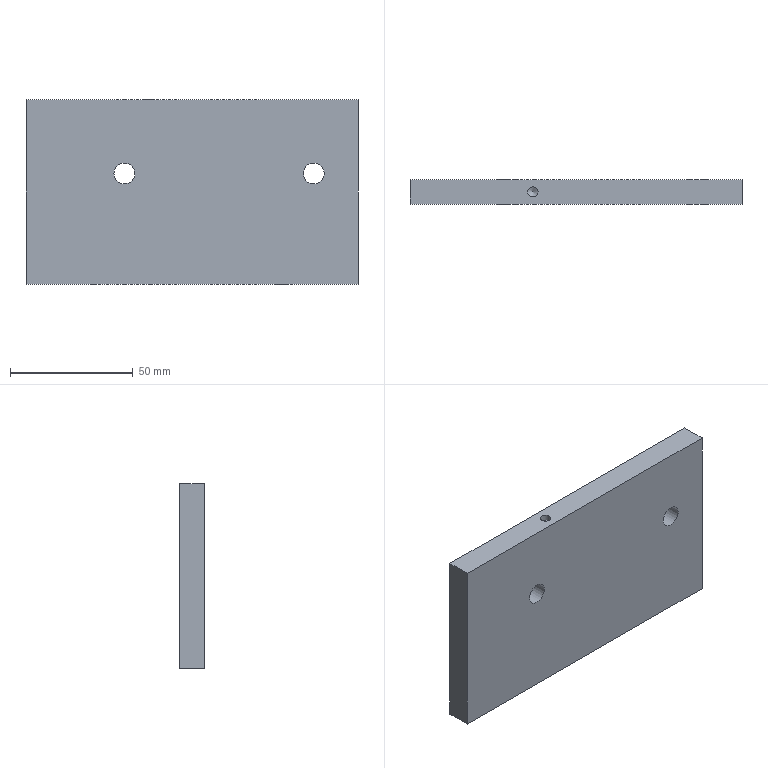Component | NX | FIXED_PLATE_15 | 1 solid | 14 faces | box 135 x 10 x 75 mm | volume 97868 mm3 | plane 6 | cylinder 5 | cone 3 | commonest cylinder face diameters 8.5 x2 6.8 x2 4.2 x1
STEP:
#1=CARTESIAN_POINT('',(0.,0.,0.));
#2=DIRECTION('',(0.,0.,1.));
#3=DIRECTION('',(1.,0.,0.));
#4=AXIS2_PLACEMENT_3D('',#1,#2,#3);
#5=CARTESIAN_POINT('',(1334.254,1421.,706.574));
#6=VERTEX_POINT('',#5);
#7=CARTESIAN_POINT('',(1334.254,1421.,781.574));
#8=VERTEX_POINT('',#7);
#9=CARTESIAN_POINT('',(1334.254,1421.,706.574));
#10=DIRECTION('',(0.,0.,1.));
#11=VECTOR('',#10,1.);
#12=LINE('',#9,#11);
#13=CARTESIAN_POINT('',(1334.254,1431.,706.574));
#14=DIRECTION('',(1.,0.,0.));
#15=DIRECTION('',(0.,0.,-1.));
#16=AXIS2_PLACEMENT_3D('',#13,#14,#15);
#17=PLANE('',#16);
#18=CARTESIAN_POINT('',(0.,-10.));
#19=DIRECTION('',(-1.,0.));
#20=VECTOR('',#19,1.);
#21=LINE('',#18,#20);
#22=(GEOMETRIC_REPRESENTATION_CONTEXT(2)PARAMETRIC_REPRESENTATION_CONTEXT()REPRESENTATION_CONTEXT('',''));
#23=DEFINITIONAL_REPRESENTATION('',(#21),#22);
#24=PCURVE('',#17,#23);
#25=CARTESIAN_POINT('',(1374.254,1421.,751.574));
#26=DIRECTION('',(0.,1.,0.));
#27=DIRECTION('',(0.,0.,1.));
#28=AXIS2_PLACEMENT_3D('',#25,#26,#27);
#29=PLANE('',#28);
#30=CARTESIAN_POINT('',(-45.,-40.));
#31=DIRECTION('',(1.,0.));
#32=VECTOR('',#31,1.);
#33=LINE('',#30,#32);
#34=(GEOMETRIC_REPRESENTATION_CONTEXT(2)PARAMETRIC_REPRESENTATION_CONTEXT()REPRESENTATION_CONTEXT('',''));
#35=DEFINITIONAL_REPRESENTATION('',(#33),#34);
#36=PCURVE('',#29,#35);
#37=SURFACE_CURVE('',#12,(#24,#36),.PCURVE_S1.);
#38=EDGE_CURVE('',#6,#8,#37,.T.);
#39=ORIENTED_EDGE('',*,*,#38,.T.);
#40=CARTESIAN_POINT('',(1334.254,1431.,781.574));
#41=VERTEX_POINT('',#40);
#42=CARTESIAN_POINT('',(1334.254,1431.,781.574));
#43=DIRECTION('',(0.,-1.,0.));
#44=VECTOR('',#43,1.);
#45=LINE('',#42,#44);
#46=CARTESIAN_POINT('',(-75.,0.));
#47=DIRECTION('',(0.,-1.));
#48=VECTOR('',#47,1.);
#49=LINE('',#46,#48);
#50=(GEOMETRIC_REPRESENTATION_CONTEXT(2)PARAMETRIC_REPRESENTATION_CONTEXT()REPRESENTATION_CONTEXT('',''));
#51=DEFINITIONAL_REPRESENTATION('',(#49),#50);
#52=PCURVE('',#17,#51);
#53=CARTESIAN_POINT('',(1334.254,1431.,781.574));
#54=DIRECTION('',(0.,0.,-1.));
#55=DIRECTION('',(-1.,0.,-0.));
#56=AXIS2_PLACEMENT_3D('',#53,#54,#55);
#57=PLANE('',#56);
#58=CARTESIAN_POINT('',(0.,0.));
#59=DIRECTION('',(0.,-1.));
#60=VECTOR('',#59,1.);
#61=LINE('',#58,#60);
#62=(GEOMETRIC_REPRESENTATION_CONTEXT(2)PARAMETRIC_REPRESENTATION_CONTEXT()REPRESENTATION_CONTEXT('',''));
#63=DEFINITIONAL_REPRESENTATION('',(#61),#62);
#64=PCURVE('',#57,#63);
#65=SURFACE_CURVE('',#45,(#52,#64),.PCURVE_S1.);
#66=EDGE_CURVE('',#41,#8,#65,.T.);
#67=ORIENTED_EDGE('',*,*,#66,.F.);
#68=CARTESIAN_POINT('',(1334.254,1431.,706.574));
#69=VERTEX_POINT('',#68);
#70=CARTESIAN_POINT('',(1334.254,1431.,706.574));
#71=DIRECTION('',(0.,0.,1.));
#72=VECTOR('',#71,1.);
#73=LINE('',#70,#72);
#74=CARTESIAN_POINT('',(0.,0.));
#75=DIRECTION('',(-1.,0.));
#76=VECTOR('',#75,1.);
#77=LINE('',#74,#76);
#78=(GEOMETRIC_REPRESENTATION_CONTEXT(2)PARAMETRIC_REPRESENTATION_CONTEXT()REPRESENTATION_CONTEXT('',''));
#79=DEFINITIONAL_REPRESENTATION('',(#77),#78);
#80=PCURVE('',#17,#79);
#81=CARTESIAN_POINT('',(1374.254,1431.,751.574));
#82=DIRECTION('',(0.,1.,0.));
#83=DIRECTION('',(0.,0.,1.));
#84=AXIS2_PLACEMENT_3D('',#81,#82,#83);
#85=PLANE('',#84);
#86=CARTESIAN_POINT('',(-45.,-40.));
#87=DIRECTION('',(1.,0.));
#88=VECTOR('',#87,1.);
#89=LINE('',#86,#88);
#90=(GEOMETRIC_REPRESENTATION_CONTEXT(2)PARAMETRIC_REPRESENTATION_CONTEXT()REPRESENTATION_CONTEXT('',''));
#91=DEFINITIONAL_REPRESENTATION('',(#89),#90);
#92=PCURVE('',#85,#91);
#93=SURFACE_CURVE('',#73,(#80,#92),.PCURVE_S1.);
#94=EDGE_CURVE('',#69,#41,#93,.T.);
#95=ORIENTED_EDGE('',*,*,#94,.F.);
#96=CARTESIAN_POINT('',(1334.254,1431.,706.574));
#97=DIRECTION('',(0.,-1.,0.));
#98=VECTOR('',#97,1.);
#99=LINE('',#96,#98);
#100=CARTESIAN_POINT('',(0.,0.));
#101=DIRECTION('',(0.,-1.));
#102=VECTOR('',#101,1.);
#103=LINE('',#100,#102);
#104=(GEOMETRIC_REPRESENTATION_CONTEXT(2)PARAMETRIC_REPRESENTATION_CONTEXT()REPRESENTATION_CONTEXT('',''));
#105=DEFINITIONAL_REPRESENTATION('',(#103),#104);
#106=PCURVE('',#17,#105);
#107=CARTESIAN_POINT('',(1469.254,1431.,706.574));
#108=DIRECTION('',(0.,0.,1.));
#109=DIRECTION('',(1.,0.,0.));
#110=AXIS2_PLACEMENT_3D('',#107,#108,#109);
#111=PLANE('',#110);
#112=CARTESIAN_POINT('',(-135.,0.));
#113=DIRECTION('',(0.,-1.));
#114=VECTOR('',#113,1.);
#115=LINE('',#112,#114);
#116=(GEOMETRIC_REPRESENTATION_CONTEXT(2)PARAMETRIC_REPRESENTATION_CONTEXT()REPRESENTATION_CONTEXT('',''));
#117=DEFINITIONAL_REPRESENTATION('',(#115),#116);
#118=PCURVE('',#111,#117);
#119=SURFACE_CURVE('',#99,(#106,#118),.PCURVE_S1.);
#120=EDGE_CURVE('',#69,#6,#119,.T.);
#121=ORIENTED_EDGE('',*,*,#120,.T.);
#122=EDGE_LOOP('',(#39,#67,#95,#121));
#123=FACE_BOUND('',#122,.T.);
#124=ADVANCED_FACE('',(#123),#17,.F.);
#125=CARTESIAN_POINT('',(1382.154,1426.,781.574));
#126=VERTEX_POINT('',#125);
#127=CARTESIAN_POINT('',(1384.254,1426.,781.574));
#128=DIRECTION('',(0.,0.,-1.));
#129=DIRECTION('',(-1.,0.,-0.));
#130=AXIS2_PLACEMENT_3D('',#127,#128,#129);
#131=CIRCLE('',#130,2.1);
#132=CARTESIAN_POINT('',(-50.,-5.));
#133=DIRECTION('',(1.,0.));
#134=AXIS2_PLACEMENT_2D('',#132,#133);
#135=CIRCLE('',#134,2.1);
#136=(GEOMETRIC_REPRESENTATION_CONTEXT(2)PARAMETRIC_REPRESENTATION_CONTEXT()REPRESENTATION_CONTEXT('',''));
#137=DEFINITIONAL_REPRESENTATION('',(#135),#136);
#138=PCURVE('',#57,#137);
#139=CARTESIAN_POINT('',(1384.254,1426.,781.574));
#140=DIRECTION('',(0.,0.,-1.));
#141=DIRECTION('',(-1.,0.,-0.));
#142=AXIS2_PLACEMENT_3D('',#139,#140,#141);
#143=CYLINDRICAL_SURFACE('',#142,2.1);
#144=CARTESIAN_POINT('',(0.,0.));
#145=DIRECTION('',(1.,0.));
#146=VECTOR('',#145,1.);
#147=LINE('',#144,#146);
#148=(GEOMETRIC_REPRESENTATION_CONTEXT(2)PARAMETRIC_REPRESENTATION_CONTEXT()REPRESENTATION_CONTEXT('',''));
#149=DEFINITIONAL_REPRESENTATION('',(#147),#148);
#150=PCURVE('',#143,#149);
#151=SURFACE_CURVE('',#131,(#138,#150),.PCURVE_S1.);
#152=EDGE_CURVE('',#126,#126,#151,.T.);
#153=ORIENTED_EDGE('',*,*,#152,.T.);
#154=EDGE_LOOP('',(#153));
#155=FACE_BOUND('',#154,.T.);
#156=CARTESIAN_POINT('',(1469.254,1421.,781.574));
#157=VERTEX_POINT('',#156);
#158=CARTESIAN_POINT('',(1334.254,1421.,781.574));
#159=DIRECTION('',(1.,0.,0.));
#160=VECTOR('',#159,1.);
#161=LINE('',#158,#160);
#162=CARTESIAN_POINT('',(0.,-10.));
#163=DIRECTION('',(-1.,0.));
#164=VECTOR('',#163,1.);
#165=LINE('',#162,#164);
#166=(GEOMETRIC_REPRESENTATION_CONTEXT(2)PARAMETRIC_REPRESENTATION_CONTEXT()REPRESENTATION_CONTEXT('',''));
#167=DEFINITIONAL_REPRESENTATION('',(#165),#166);
#168=PCURVE('',#57,#167);
#169=CARTESIAN_POINT('',(30.,-40.));
#170=DIRECTION('',(0.,1.));
#171=VECTOR('',#170,1.);
#172=LINE('',#169,#171);
#173=(GEOMETRIC_REPRESENTATION_CONTEXT(2)PARAMETRIC_REPRESENTATION_CONTEXT()REPRESENTATION_CONTEXT('',''));
#174=DEFINITIONAL_REPRESENTATION('',(#172),#173);
#175=PCURVE('',#29,#174);
#176=SURFACE_CURVE('',#161,(#168,#175),.PCURVE_S1.);
#177=EDGE_CURVE('',#8,#157,#176,.T.);
#178=ORIENTED_EDGE('',*,*,#177,.T.);
#179=CARTESIAN_POINT('',(1469.254,1431.,781.574));
#180=VERTEX_POINT('',#179);
#181=CARTESIAN_POINT('',(1469.254,1431.,781.574));
#182=DIRECTION('',(0.,-1.,0.));
#183=VECTOR('',#182,1.);
#184=LINE('',#181,#183);
#185=CARTESIAN_POINT('',(-135.,0.));
#186=DIRECTION('',(0.,-1.));
#187=VECTOR('',#186,1.);
#188=LINE('',#185,#187);
#189=(GEOMETRIC_REPRESENTATION_CONTEXT(2)PARAMETRIC_REPRESENTATION_CONTEXT()REPRESENTATION_CONTEXT('',''));
#190=DEFINITIONAL_REPRESENTATION('',(#188),#189);
#191=PCURVE('',#57,#190);
#192=CARTESIAN_POINT('',(1469.254,1431.,781.574));
#193=DIRECTION('',(-1.,0.,0.));
#194=DIRECTION('',(0.,0.,1.));
#195=AXIS2_PLACEMENT_3D('',#192,#193,#194);
#196=PLANE('',#195);
#197=CARTESIAN_POINT('',(0.,0.));
#198=DIRECTION('',(0.,-1.));
#199=VECTOR('',#198,1.);
#200=LINE('',#197,#199);
#201=(GEOMETRIC_REPRESENTATION_CONTEXT(2)PARAMETRIC_REPRESENTATION_CONTEXT()REPRESENTATION_CONTEXT('',''));
#202=DEFINITIONAL_REPRESENTATION('',(#200),#201);
#203=PCURVE('',#196,#202);
#204=SURFACE_CURVE('',#184,(#191,#203),.PCURVE_S1.);
#205=EDGE_CURVE('',#180,#157,#204,.T.);
#206=ORIENTED_EDGE('',*,*,#205,.F.);
#207=CARTESIAN_POINT('',(1334.254,1431.,781.574));
#208=DIRECTION('',(1.,0.,0.));
#209=VECTOR('',#208,1.);
#210=LINE('',#207,#209);
#211=CARTESIAN_POINT('',(0.,0.));
#212=DIRECTION('',(-1.,0.));
#213=VECTOR('',#212,1.);
#214=LINE('',#211,#213);
#215=(GEOMETRIC_REPRESENTATION_CONTEXT(2)PARAMETRIC_REPRESENTATION_CONTEXT()REPRESENTATION_CONTEXT('',''));
#216=DEFINITIONAL_REPRESENTATION('',(#214),#215);
#217=PCURVE('',#57,#216);
#218=CARTESIAN_POINT('',(30.,-40.));
#219=DIRECTION('',(0.,1.));
#220=VECTOR('',#219,1.);
#221=LINE('',#218,#220);
#222=(GEOMETRIC_REPRESENTATION_CONTEXT(2)PARAMETRIC_REPRESENTATION_CONTEXT()REPRESENTATION_CONTEXT('',''));
#223=DEFINITIONAL_REPRESENTATION('',(#221),#222);
#224=PCURVE('',#85,#223);
#225=SURFACE_CURVE('',#210,(#217,#224),.PCURVE_S1.);
#226=EDGE_CURVE('',#41,#180,#225,.T.);
#227=ORIENTED_EDGE('',*,*,#226,.F.);
#228=ORIENTED_EDGE('',*,*,#66,.T.);
#229=EDGE_LOOP('',(#178,#206,#227,#228));
#230=FACE_BOUND('',#229,.T.);
#231=ADVANCED_FACE('',(#155,#230),#57,.F.);
#232=CARTESIAN_POINT('',(1469.254,1421.,706.574));
#233=VERTEX_POINT('',#232);
#234=CARTESIAN_POINT('',(1469.254,1421.,781.574));
#235=DIRECTION('',(0.,0.,-1.));
#236=VECTOR('',#235,1.);
#237=LINE('',#234,#236);
#238=CARTESIAN_POINT('',(0.,-10.));
#239=DIRECTION('',(-1.,0.));
#240=VECTOR('',#239,1.);
#241=LINE('',#238,#240);
#242=(GEOMETRIC_REPRESENTATION_CONTEXT(2)PARAMETRIC_REPRESENTATION_CONTEXT()REPRESENTATION_CONTEXT('',''));
#243=DEFINITIONAL_REPRESENTATION('',(#241),#242);
#244=PCURVE('',#196,#243);
#245=CARTESIAN_POINT('',(30.,95.));
#246=DIRECTION('',(-1.,0.));
#247=VECTOR('',#246,1.);
#248=LINE('',#245,#247);
#249=(GEOMETRIC_REPRESENTATION_CONTEXT(2)PARAMETRIC_REPRESENTATION_CONTEXT()REPRESENTATION_CONTEXT('',''));
#250=DEFINITIONAL_REPRESENTATION('',(#248),#249);
#251=PCURVE('',#29,#250);
#252=SURFACE_CURVE('',#237,(#244,#251),.PCURVE_S1.);
#253=EDGE_CURVE('',#157,#233,#252,.T.);
#254=ORIENTED_EDGE('',*,*,#253,.T.);
#255=CARTESIAN_POINT('',(1469.254,1431.,706.574));
#256=VERTEX_POINT('',#255);
#257=CARTESIAN_POINT('',(1469.254,1431.,706.574));
#258=DIRECTION('',(0.,-1.,0.));
#259=VECTOR('',#258,1.);
#260=LINE('',#257,#259);
#261=CARTESIAN_POINT('',(-75.,0.));
#262=DIRECTION('',(0.,-1.));
#263=VECTOR('',#262,1.);
#264=LINE('',#261,#263);
#265=(GEOMETRIC_REPRESENTATION_CONTEXT(2)PARAMETRIC_REPRESENTATION_CONTEXT()REPRESENTATION_CONTEXT('',''));
#266=DEFINITIONAL_REPRESENTATION('',(#264),#265);
#267=PCURVE('',#196,#266);
#268=CARTESIAN_POINT('',(0.,0.));
#269=DIRECTION('',(0.,-1.));
#270=VECTOR('',#269,1.);
#271=LINE('',#268,#270);
#272=(GEOMETRIC_REPRESENTATION_CONTEXT(2)PARAMETRIC_REPRESENTATION_CONTEXT()REPRESENTATION_CONTEXT('',''));
#273=DEFINITIONAL_REPRESENTATION('',(#271),#272);
#274=PCURVE('',#111,#273);
#275=SURFACE_CURVE('',#260,(#267,#274),.PCURVE_S1.);
#276=EDGE_CURVE('',#256,#233,#275,.T.);
#277=ORIENTED_EDGE('',*,*,#276,.F.);
#278=CARTESIAN_POINT('',(1469.254,1431.,781.574));
#279=DIRECTION('',(0.,0.,-1.));
#280=VECTOR('',#279,1.);
#281=LINE('',#278,#280);
#282=CARTESIAN_POINT('',(0.,0.));
#283=DIRECTION('',(-1.,0.));
#284=VECTOR('',#283,1.);
#285=LINE('',#282,#284);
#286=(GEOMETRIC_REPRESENTATION_CONTEXT(2)PARAMETRIC_REPRESENTATION_CONTEXT()REPRESENTATION_CONTEXT('',''));
#287=DEFINITIONAL_REPRESENTATION('',(#285),#286);
#288=PCURVE('',#196,#287);
#289=CARTESIAN_POINT('',(30.,95.));
#290=DIRECTION('',(-1.,0.));
#291=VECTOR('',#290,1.);
#292=LINE('',#289,#291);
#293=(GEOMETRIC_REPRESENTATION_CONTEXT(2)PARAMETRIC_REPRESENTATION_CONTEXT()REPRESENTATION_CONTEXT('',''));
#294=DEFINITIONAL_REPRESENTATION('',(#292),#293);
#295=PCURVE('',#85,#294);
#296=SURFACE_CURVE('',#281,(#288,#295),.PCURVE_S1.);
#297=EDGE_CURVE('',#180,#256,#296,.T.);
#298=ORIENTED_EDGE('',*,*,#297,.F.);
#299=ORIENTED_EDGE('',*,*,#205,.T.);
#300=EDGE_LOOP('',(#254,#277,#298,#299));
#301=FACE_BOUND('',#300,.T.);
#302=ADVANCED_FACE('',(#301),#196,.F.);
#303=CARTESIAN_POINT('',(1378.504,1431.,751.574));
#304=VERTEX_POINT('',#303);
#305=CARTESIAN_POINT('',(1374.254,1431.,751.574));
#306=DIRECTION('',(0.,1.,0.));
#307=DIRECTION('',(1.,0.,0.));
#308=AXIS2_PLACEMENT_3D('',#305,#306,#307);
#309=CIRCLE('',#308,4.25);
#310=CARTESIAN_POINT('',(1374.254,1431.,751.574));
#311=DIRECTION('',(0.,-1.,0.));
#312=DIRECTION('',(0.,0.,-1.));
#313=AXIS2_PLACEMENT_3D('',#310,#311,#312);
#314=CYLINDRICAL_SURFACE('',#313,4.25);
#315=CARTESIAN_POINT('',(7.854,0.));
#316=DIRECTION('',(-1.,0.));
#317=VECTOR('',#316,1.);
#318=LINE('',#315,#317);
#319=(GEOMETRIC_REPRESENTATION_CONTEXT(2)PARAMETRIC_REPRESENTATION_CONTEXT()REPRESENTATION_CONTEXT('',''));
#320=DEFINITIONAL_REPRESENTATION('',(#318),#319);
#321=PCURVE('',#314,#320);
#322=CARTESIAN_POINT('',(0.,0.));
#323=DIRECTION('',(0.,1.));
#324=AXIS2_PLACEMENT_2D('',#322,#323);
#325=CIRCLE('',#324,4.25);
#326=(GEOMETRIC_REPRESENTATION_CONTEXT(2)PARAMETRIC_REPRESENTATION_CONTEXT()REPRESENTATION_CONTEXT('',''));
#327=DEFINITIONAL_REPRESENTATION('',(#325),#326);
#328=PCURVE('',#85,#327);
#329=SURFACE_CURVE('',#309,(#321,#328),.PCURVE_S1.);
#330=EDGE_CURVE('',#304,#304,#329,.T.);
#331=ORIENTED_EDGE('',*,*,#330,.F.);
#332=CARTESIAN_POINT('',(1378.504,1421.,751.574));
#333=VERTEX_POINT('',#332);
#334=CARTESIAN_POINT('',(1378.504,1431.,751.574));
#335=CARTESIAN_POINT('',(1378.504,1421.,751.574));
#336=B_SPLINE_CURVE_WITH_KNOTS('',1,(#334,#335),.UNSPECIFIED.,.F.,.F.,(2,2),(0.,10.),.PIECEWISE_BEZIER_KNOTS.);
#337=CARTESIAN_POINT('',(7.854,0.));
#338=DIRECTION('',(0.,1.));
#339=VECTOR('',#338,1.);
#340=LINE('',#337,#339);
#341=(GEOMETRIC_REPRESENTATION_CONTEXT(2)PARAMETRIC_REPRESENTATION_CONTEXT()REPRESENTATION_CONTEXT('',''));
#342=DEFINITIONAL_REPRESENTATION('',(#340),#341);
#343=PCURVE('',#314,#342);
#344=CARTESIAN_POINT('',(1.571,0.));
#345=DIRECTION('',(0.,1.));
#346=VECTOR('',#345,1.);
#347=LINE('',#344,#346);
#348=(GEOMETRIC_REPRESENTATION_CONTEXT(2)PARAMETRIC_REPRESENTATION_CONTEXT()REPRESENTATION_CONTEXT('',''));
#349=DEFINITIONAL_REPRESENTATION('',(#347),#348);
#350=PCURVE('',#314,#349);
#351=SEAM_CURVE('',#336,(#343,#350),.PCURVE_S1.);
#352=EDGE_CURVE('',#304,#333,#351,.T.);
#353=ORIENTED_EDGE('',*,*,#352,.T.);
#354=CARTESIAN_POINT('',(1374.254,1421.,751.574));
#355=DIRECTION('',(0.,1.,0.));
#356=DIRECTION('',(1.,0.,0.));
#357=AXIS2_PLACEMENT_3D('',#354,#355,#356);
#358=CIRCLE('',#357,4.25);
#359=CARTESIAN_POINT('',(7.854,10.));
#360=DIRECTION('',(-1.,0.));
#361=VECTOR('',#360,1.);
#362=LINE('',#359,#361);
#363=(GEOMETRIC_REPRESENTATION_CONTEXT(2)PARAMETRIC_REPRESENTATION_CONTEXT()REPRESENTATION_CONTEXT('',''));
#364=DEFINITIONAL_REPRESENTATION('',(#362),#363);
#365=PCURVE('',#314,#364);
#366=CARTESIAN_POINT('',(0.,0.));
#367=DIRECTION('',(0.,1.));
#368=AXIS2_PLACEMENT_2D('',#366,#367);
#369=CIRCLE('',#368,4.25);
#370=(GEOMETRIC_REPRESENTATION_CONTEXT(2)PARAMETRIC_REPRESENTATION_CONTEXT()REPRESENTATION_CONTEXT('',''));
#371=DEFINITIONAL_REPRESENTATION('',(#369),#370);
#372=PCURVE('',#29,#371);
#373=SURFACE_CURVE('',#358,(#365,#372),.PCURVE_S1.);
#374=EDGE_CURVE('',#333,#333,#373,.T.);
#375=ORIENTED_EDGE('',*,*,#374,.T.);
#376=ORIENTED_EDGE('',*,*,#352,.F.);
#377=EDGE_LOOP('',(#331,#353,#375,#376));
#378=FACE_BOUND('',#377,.F.);
#379=ADVANCED_FACE('',(#378),#314,.F.);
#380=CARTESIAN_POINT('',(1442.654,1427.,706.574));
#381=VERTEX_POINT('',#380);
#382=CARTESIAN_POINT('',(1439.254,1427.,706.574));
#383=DIRECTION('',(0.,0.,1.));
#384=DIRECTION('',(1.,0.,0.));
#385=AXIS2_PLACEMENT_3D('',#382,#383,#384);
#386=CIRCLE('',#385,3.4);
#387=CARTESIAN_POINT('',(-30.,-4.));
#388=DIRECTION('',(1.,0.));
#389=AXIS2_PLACEMENT_2D('',#387,#388);
#390=CIRCLE('',#389,3.4);
#391=(GEOMETRIC_REPRESENTATION_CONTEXT(2)PARAMETRIC_REPRESENTATION_CONTEXT()REPRESENTATION_CONTEXT('',''));
#392=DEFINITIONAL_REPRESENTATION('',(#390),#391);
#393=PCURVE('',#111,#392);
#394=CARTESIAN_POINT('',(1439.254,1427.,706.574));
#395=DIRECTION('',(0.,0.,1.));
#396=DIRECTION('',(1.,0.,0.));
#397=AXIS2_PLACEMENT_3D('',#394,#395,#396);
#398=CYLINDRICAL_SURFACE('',#397,3.4);
#399=CARTESIAN_POINT('',(0.,0.));
#400=DIRECTION('',(1.,0.));
#401=VECTOR('',#400,1.);
#402=LINE('',#399,#401);
#403=(GEOMETRIC_REPRESENTATION_CONTEXT(2)PARAMETRIC_REPRESENTATION_CONTEXT()REPRESENTATION_CONTEXT('',''));
#404=DEFINITIONAL_REPRESENTATION('',(#402),#403);
#405=PCURVE('',#398,#404);
#406=SURFACE_CURVE('',#386,(#393,#405),.PCURVE_S1.);
#407=EDGE_CURVE('',#381,#381,#406,.T.);
#408=ORIENTED_EDGE('',*,*,#407,.T.);
#409=EDGE_LOOP('',(#408));
#410=FACE_BOUND('',#409,.T.);
#411=CARTESIAN_POINT('',(1367.654,1427.,706.574));
#412=VERTEX_POINT('',#411);
#413=CARTESIAN_POINT('',(1364.254,1427.,706.574));
#414=DIRECTION('',(0.,0.,1.));
#415=DIRECTION('',(1.,0.,0.));
#416=AXIS2_PLACEMENT_3D('',#413,#414,#415);
#417=CIRCLE('',#416,3.4);
#418=CARTESIAN_POINT('',(-105.,-4.));
#419=DIRECTION('',(1.,0.));
#420=AXIS2_PLACEMENT_2D('',#418,#419);
#421=CIRCLE('',#420,3.4);
#422=(GEOMETRIC_REPRESENTATION_CONTEXT(2)PARAMETRIC_REPRESENTATION_CONTEXT()REPRESENTATION_CONTEXT('',''));
#423=DEFINITIONAL_REPRESENTATION('',(#421),#422);
#424=PCURVE('',#111,#423);
#425=CARTESIAN_POINT('',(1364.254,1427.,706.574));
#426=DIRECTION('',(0.,0.,1.));
#427=DIRECTION('',(1.,0.,0.));
#428=AXIS2_PLACEMENT_3D('',#425,#426,#427);
#429=CYLINDRICAL_SURFACE('',#428,3.4);
#430=CARTESIAN_POINT('',(0.,0.));
#431=DIRECTION('',(1.,0.));
#432=VECTOR('',#431,1.);
#433=LINE('',#430,#432);
#434=(GEOMETRIC_REPRESENTATION_CONTEXT(2)PARAMETRIC_REPRESENTATION_CONTEXT()REPRESENTATION_CONTEXT('',''));
#435=DEFINITIONAL_REPRESENTATION('',(#433),#434);
#436=PCURVE('',#429,#435);
#437=SURFACE_CURVE('',#417,(#424,#436),.PCURVE_S1.);
#438=EDGE_CURVE('',#412,#412,#437,.T.);
#439=ORIENTED_EDGE('',*,*,#438,.T.);
#440=EDGE_LOOP('',(#439));
#441=FACE_BOUND('',#440,.T.);
#442=CARTESIAN_POINT('',(1469.254,1421.,706.574));
#443=DIRECTION('',(-1.,0.,0.));
#444=VECTOR('',#443,1.);
#445=LINE('',#442,#444);
#446=CARTESIAN_POINT('',(0.,-10.));
#447=DIRECTION('',(-1.,0.));
#448=VECTOR('',#447,1.);
#449=LINE('',#446,#448);
#450=(GEOMETRIC_REPRESENTATION_CONTEXT(2)PARAMETRIC_REPRESENTATION_CONTEXT()REPRESENTATION_CONTEXT('',''));
#451=DEFINITIONAL_REPRESENTATION('',(#449),#450);
#452=PCURVE('',#111,#451);
#453=CARTESIAN_POINT('',(-45.,95.));
#454=DIRECTION('',(0.,-1.));
#455=VECTOR('',#454,1.);
#456=LINE('',#453,#455);
#457=(GEOMETRIC_REPRESENTATION_CONTEXT(2)PARAMETRIC_REPRESENTATION_CONTEXT()REPRESENTATION_CONTEXT('',''));
#458=DEFINITIONAL_REPRESENTATION('',(#456),#457);
#459=PCURVE('',#29,#458);
#460=SURFACE_CURVE('',#445,(#452,#459),.PCURVE_S1.);
#461=EDGE_CURVE('',#233,#6,#460,.T.);
#462=ORIENTED_EDGE('',*,*,#461,.T.);
#463=ORIENTED_EDGE('',*,*,#120,.F.);
#464=CARTESIAN_POINT('',(1469.254,1431.,706.574));
#465=DIRECTION('',(-1.,0.,0.));
#466=VECTOR('',#465,1.);
#467=LINE('',#464,#466);
#468=CARTESIAN_POINT('',(0.,0.));
#469=DIRECTION('',(-1.,0.));
#470=VECTOR('',#469,1.);
#471=LINE('',#468,#470);
#472=(GEOMETRIC_REPRESENTATION_CONTEXT(2)PARAMETRIC_REPRESENTATION_CONTEXT()REPRESENTATION_CONTEXT('',''));
#473=DEFINITIONAL_REPRESENTATION('',(#471),#472);
#474=PCURVE('',#111,#473);
#475=CARTESIAN_POINT('',(-45.,95.));
#476=DIRECTION('',(0.,-1.));
#477=VECTOR('',#476,1.);
#478=LINE('',#475,#477);
#479=(GEOMETRIC_REPRESENTATION_CONTEXT(2)PARAMETRIC_REPRESENTATION_CONTEXT()REPRESENTATION_CONTEXT('',''));
#480=DEFINITIONAL_REPRESENTATION('',(#478),#479);
#481=PCURVE('',#85,#480);
#482=SURFACE_CURVE('',#467,(#474,#481),.PCURVE_S1.);
#483=EDGE_CURVE('',#256,#69,#482,.T.);
#484=ORIENTED_EDGE('',*,*,#483,.F.);
#485=ORIENTED_EDGE('',*,*,#276,.T.);
#486=EDGE_LOOP('',(#462,#463,#484,#485));
#487=FACE_BOUND('',#486,.T.);
#488=ADVANCED_FACE('',(#410,#441,#487),#111,.F.);
#489=CARTESIAN_POINT('',(1455.504,1431.,751.574));
#490=VERTEX_POINT('',#489);
#491=CARTESIAN_POINT('',(1451.254,1431.,751.574));
#492=DIRECTION('',(0.,1.,0.));
#493=DIRECTION('',(1.,0.,0.));
#494=AXIS2_PLACEMENT_3D('',#491,#492,#493);
#495=CIRCLE('',#494,4.25);
#496=CARTESIAN_POINT('',(1451.254,1431.,751.574));
#497=DIRECTION('',(0.,-1.,0.));
#498=DIRECTION('',(0.,0.,-1.));
#499=AXIS2_PLACEMENT_3D('',#496,#497,#498);
#500=CYLINDRICAL_SURFACE('',#499,4.25);
#501=CARTESIAN_POINT('',(7.854,0.));
#502=DIRECTION('',(-1.,0.));
#503=VECTOR('',#502,1.);
#504=LINE('',#501,#503);
#505=(GEOMETRIC_REPRESENTATION_CONTEXT(2)PARAMETRIC_REPRESENTATION_CONTEXT()REPRESENTATION_CONTEXT('',''));
#506=DEFINITIONAL_REPRESENTATION('',(#504),#505);
#507=PCURVE('',#500,#506);
#508=CARTESIAN_POINT('',(0.,77.));
#509=DIRECTION('',(0.,1.));
#510=AXIS2_PLACEMENT_2D('',#508,#509);
#511=CIRCLE('',#510,4.25);
#512=(GEOMETRIC_REPRESENTATION_CONTEXT(2)PARAMETRIC_REPRESENTATION_CONTEXT()REPRESENTATION_CONTEXT('',''));
#513=DEFINITIONAL_REPRESENTATION('',(#511),#512);
#514=PCURVE('',#85,#513);
#515=SURFACE_CURVE('',#495,(#507,#514),.PCURVE_S1.);
#516=EDGE_CURVE('',#490,#490,#515,.T.);
#517=ORIENTED_EDGE('',*,*,#516,.F.);
#518=CARTESIAN_POINT('',(1455.504,1421.,751.574));
#519=VERTEX_POINT('',#518);
#520=CARTESIAN_POINT('',(1455.504,1431.,751.574));
#521=CARTESIAN_POINT('',(1455.504,1421.,751.574));
#522=B_SPLINE_CURVE_WITH_KNOTS('',1,(#520,#521),.UNSPECIFIED.,.F.,.F.,(2,2),(0.,10.),.PIECEWISE_BEZIER_KNOTS.);
#523=CARTESIAN_POINT('',(7.854,0.));
#524=DIRECTION('',(0.,1.));
#525=VECTOR('',#524,1.);
#526=LINE('',#523,#525);
#527=(GEOMETRIC_REPRESENTATION_CONTEXT(2)PARAMETRIC_REPRESENTATION_CONTEXT()REPRESENTATION_CONTEXT('',''));
#528=DEFINITIONAL_REPRESENTATION('',(#526),#527);
#529=PCURVE('',#500,#528);
#530=CARTESIAN_POINT('',(1.571,0.));
#531=DIRECTION('',(0.,1.));
#532=VECTOR('',#531,1.);
#533=LINE('',#530,#532);
#534=(GEOMETRIC_REPRESENTATION_CONTEXT(2)PARAMETRIC_REPRESENTATION_CONTEXT()REPRESENTATION_CONTEXT('',''));
#535=DEFINITIONAL_REPRESENTATION('',(#533),#534);
#536=PCURVE('',#500,#535);
#537=SEAM_CURVE('',#522,(#529,#536),.PCURVE_S1.);
#538=EDGE_CURVE('',#490,#519,#537,.T.);
#539=ORIENTED_EDGE('',*,*,#538,.T.);
#540=CARTESIAN_POINT('',(1451.254,1421.,751.574));
#541=DIRECTION('',(0.,1.,0.));
#542=DIRECTION('',(1.,0.,0.));
#543=AXIS2_PLACEMENT_3D('',#540,#541,#542);
#544=CIRCLE('',#543,4.25);
#545=CARTESIAN_POINT('',(7.854,10.));
#546=DIRECTION('',(-1.,0.));
#547=VECTOR('',#546,1.);
#548=LINE('',#545,#547);
#549=(GEOMETRIC_REPRESENTATION_CONTEXT(2)PARAMETRIC_REPRESENTATION_CONTEXT()REPRESENTATION_CONTEXT('',''));
#550=DEFINITIONAL_REPRESENTATION('',(#548),#549);
#551=PCURVE('',#500,#550);
#552=CARTESIAN_POINT('',(0.,77.));
#553=DIRECTION('',(0.,1.));
#554=AXIS2_PLACEMENT_2D('',#552,#553);
#555=CIRCLE('',#554,4.25);
#556=(GEOMETRIC_REPRESENTATION_CONTEXT(2)PARAMETRIC_REPRESENTATION_CONTEXT()REPRESENTATION_CONTEXT('',''));
#557=DEFINITIONAL_REPRESENTATION('',(#555),#556);
#558=PCURVE('',#29,#557);
#559=SURFACE_CURVE('',#544,(#551,#558),.PCURVE_S1.);
#560=EDGE_CURVE('',#519,#519,#559,.T.);
#561=ORIENTED_EDGE('',*,*,#560,.T.);
#562=ORIENTED_EDGE('',*,*,#538,.F.);
#563=EDGE_LOOP('',(#517,#539,#561,#562));
#564=FACE_BOUND('',#563,.F.);
#565=ADVANCED_FACE('',(#564),#500,.F.);
#566=ORIENTED_EDGE('',*,*,#94,.T.);
#567=ORIENTED_EDGE('',*,*,#226,.T.);
#568=ORIENTED_EDGE('',*,*,#297,.T.);
#569=ORIENTED_EDGE('',*,*,#483,.T.);
#570=EDGE_LOOP('',(#566,#567,#568,#569));
#571=FACE_BOUND('',#570,.T.);
#572=ORIENTED_EDGE('',*,*,#330,.F.);
#573=EDGE_LOOP('',(#572));
#574=FACE_BOUND('',#573,.T.);
#575=ORIENTED_EDGE('',*,*,#516,.F.);
#576=EDGE_LOOP('',(#575));
#577=FACE_BOUND('',#576,.T.);
#578=ADVANCED_FACE('',(#571,#574,#577),#85,.T.);
#579=ORIENTED_EDGE('',*,*,#38,.F.);
#580=ORIENTED_EDGE('',*,*,#461,.F.);
#581=ORIENTED_EDGE('',*,*,#253,.F.);
#582=ORIENTED_EDGE('',*,*,#177,.F.);
#583=EDGE_LOOP('',(#579,#580,#581,#582));
#584=FACE_BOUND('',#583,.T.);
#585=ORIENTED_EDGE('',*,*,#374,.T.);
#586=EDGE_LOOP('',(#585));
#587=FACE_BOUND('',#586,.T.);
#588=ORIENTED_EDGE('',*,*,#560,.T.);
#589=EDGE_LOOP('',(#588));
#590=FACE_BOUND('',#589,.T.);
#591=ADVANCED_FACE('',(#584,#587,#590),#29,.F.);
#592=CARTESIAN_POINT('',(1386.354,1426.,779.174));
#593=VERTEX_POINT('',#592);
#594=CARTESIAN_POINT('',(1382.154,1426.,779.174));
#595=VERTEX_POINT('',#594);
#596=CARTESIAN_POINT('',(1384.254,1426.,779.174));
#597=DIRECTION('',(-0.,0.,1.));
#598=DIRECTION('',(-1.,0.,-0.));
#599=AXIS2_PLACEMENT_3D('',#596,#597,#598);
#600=CIRCLE('',#599,2.1);
#601=CARTESIAN_POINT('',(1384.254,1426.,779.174));
#602=DIRECTION('',(-0.,0.,1.));
#603=DIRECTION('',(1.,0.,0.));
#604=AXIS2_PLACEMENT_3D('',#601,#602,#603);
#605=CONICAL_SURFACE('',#604,2.1,1.047);
#606=CARTESIAN_POINT('',(-3.142,-0.));
#607=DIRECTION('',(1.,0.));
#608=VECTOR('',#607,1.);
#609=LINE('',#606,#608);
#610=(GEOMETRIC_REPRESENTATION_CONTEXT(2)PARAMETRIC_REPRESENTATION_CONTEXT()REPRESENTATION_CONTEXT('',''));
#611=DEFINITIONAL_REPRESENTATION('',(#609),#610);
#612=PCURVE('',#605,#611);
#613=CARTESIAN_POINT('',(6.283,2.4));
#614=DIRECTION('',(-1.,0.));
#615=VECTOR('',#614,1.);
#616=LINE('',#613,#615);
#617=(GEOMETRIC_REPRESENTATION_CONTEXT(2)PARAMETRIC_REPRESENTATION_CONTEXT()REPRESENTATION_CONTEXT('',''));
#618=DEFINITIONAL_REPRESENTATION('',(#616),#617);
#619=PCURVE('',#143,#618);
#620=SURFACE_CURVE('',#600,(#612,#619),.PCURVE_S1.);
#621=EDGE_CURVE('',#593,#595,#620,.T.);
#622=ORIENTED_EDGE('',*,*,#621,.F.);
#623=CARTESIAN_POINT('',(1384.254,1426.,777.961));
#624=VERTEX_POINT('',#623);
#625=CARTESIAN_POINT('',(1384.254,1426.,777.961));
#626=CARTESIAN_POINT('',(1386.354,1426.,779.174));
#627=B_SPLINE_CURVE_WITH_KNOTS('',1,(#625,#626),.UNSPECIFIED.,.F.,.F.,(2,2),(-2.425,-0.),.PIECEWISE_BEZIER_KNOTS.);
#628=CARTESIAN_POINT('',(0.,0.));
#629=DIRECTION('',(0.,1.));
#630=VECTOR('',#629,1.);
#631=LINE('',#628,#630);
#632=(GEOMETRIC_REPRESENTATION_CONTEXT(2)PARAMETRIC_REPRESENTATION_CONTEXT()REPRESENTATION_CONTEXT('',''));
#633=DEFINITIONAL_REPRESENTATION('',(#631),#632);
#634=PCURVE('',#605,#633);
#635=CARTESIAN_POINT('',(6.283,0.));
#636=DIRECTION('',(0.,1.));
#637=VECTOR('',#636,1.);
#638=LINE('',#635,#637);
#639=(GEOMETRIC_REPRESENTATION_CONTEXT(2)PARAMETRIC_REPRESENTATION_CONTEXT()REPRESENTATION_CONTEXT('',''));
#640=DEFINITIONAL_REPRESENTATION('',(#638),#639);
#641=PCURVE('',#605,#640);
#642=SEAM_CURVE('',#627,(#634,#641),.PCURVE_S1.);
#643=EDGE_CURVE('',#624,#593,#642,.T.);
#644=ORIENTED_EDGE('',*,*,#643,.F.);
#645=ORIENTED_EDGE('',*,*,#643,.T.);
#646=CARTESIAN_POINT('',(1384.254,1426.,779.174));
#647=DIRECTION('',(-0.,0.,1.));
#648=DIRECTION('',(-1.,0.,-0.));
#649=AXIS2_PLACEMENT_3D('',#646,#647,#648);
#650=CIRCLE('',#649,2.1);
#651=CARTESIAN_POINT('',(3.142,-0.));
#652=DIRECTION('',(1.,0.));
#653=VECTOR('',#652,1.);
#654=LINE('',#651,#653);
#655=(GEOMETRIC_REPRESENTATION_CONTEXT(2)PARAMETRIC_REPRESENTATION_CONTEXT()REPRESENTATION_CONTEXT('',''));
#656=DEFINITIONAL_REPRESENTATION('',(#654),#655);
#657=PCURVE('',#605,#656);
#658=CARTESIAN_POINT('',(6.283,2.4));
#659=DIRECTION('',(-1.,0.));
#660=VECTOR('',#659,1.);
#661=LINE('',#658,#660);
#662=(GEOMETRIC_REPRESENTATION_CONTEXT(2)PARAMETRIC_REPRESENTATION_CONTEXT()REPRESENTATION_CONTEXT('',''));
#663=DEFINITIONAL_REPRESENTATION('',(#661),#662);
#664=PCURVE('',#143,#663);
#665=SURFACE_CURVE('',#650,(#657,#664),.PCURVE_S1.);
#666=EDGE_CURVE('',#595,#593,#665,.T.);
#667=ORIENTED_EDGE('',*,*,#666,.F.);
#668=EDGE_LOOP('',(#622,#644,#645,#667));
#669=FACE_BOUND('',#668,.F.);
#670=ADVANCED_FACE('',(#669),#605,.F.);
#671=ORIENTED_EDGE('',*,*,#621,.T.);
#672=CARTESIAN_POINT('',(1382.154,1426.,781.574));
#673=CARTESIAN_POINT('',(1382.154,1426.,779.174));
#674=B_SPLINE_CURVE_WITH_KNOTS('',1,(#672,#673),.UNSPECIFIED.,.F.,.F.,(2,2),(0.,2.4),.PIECEWISE_BEZIER_KNOTS.);
#675=CARTESIAN_POINT('',(0.,0.));
#676=DIRECTION('',(0.,1.));
#677=VECTOR('',#676,1.);
#678=LINE('',#675,#677);
#679=(GEOMETRIC_REPRESENTATION_CONTEXT(2)PARAMETRIC_REPRESENTATION_CONTEXT()REPRESENTATION_CONTEXT('',''));
#680=DEFINITIONAL_REPRESENTATION('',(#678),#679);
#681=PCURVE('',#143,#680);
#682=CARTESIAN_POINT('',(6.283,0.));
#683=DIRECTION('',(0.,1.));
#684=VECTOR('',#683,1.);
#685=LINE('',#682,#684);
#686=(GEOMETRIC_REPRESENTATION_CONTEXT(2)PARAMETRIC_REPRESENTATION_CONTEXT()REPRESENTATION_CONTEXT('',''));
#687=DEFINITIONAL_REPRESENTATION('',(#685),#686);
#688=PCURVE('',#143,#687);
#689=SEAM_CURVE('',#674,(#681,#688),.PCURVE_S1.);
#690=EDGE_CURVE('',#126,#595,#689,.T.);
#691=ORIENTED_EDGE('',*,*,#690,.F.);
#692=ORIENTED_EDGE('',*,*,#152,.T.);
#693=ORIENTED_EDGE('',*,*,#690,.T.);
#694=ORIENTED_EDGE('',*,*,#666,.T.);
#695=EDGE_LOOP('',(#671,#691,#692,#693,#694));
#696=FACE_BOUND('',#695,.F.);
#697=ADVANCED_FACE('',(#696),#143,.F.);
#698=CARTESIAN_POINT('',(1360.854,1427.,736.324));
#699=VERTEX_POINT('',#698);
#700=CARTESIAN_POINT('',(1367.654,1427.,736.324));
#701=VERTEX_POINT('',#700);
#702=CARTESIAN_POINT('',(1364.254,1427.,736.324));
#703=DIRECTION('',(0.,0.,-1.));
#704=DIRECTION('',(1.,0.,0.));
#705=AXIS2_PLACEMENT_3D('',#702,#703,#704);
#706=CIRCLE('',#705,3.4);
#707=CARTESIAN_POINT('',(1364.254,1427.,736.324));
#708=DIRECTION('',(0.,0.,-1.));
#709=DIRECTION('',(-1.,0.,0.));
#710=AXIS2_PLACEMENT_3D('',#707,#708,#709);
#711=CONICAL_SURFACE('',#710,3.4,1.047);
#712=CARTESIAN_POINT('',(-3.142,0.));
#713=DIRECTION('',(1.,0.));
#714=VECTOR('',#713,1.);
#715=LINE('',#712,#714);
#716=(GEOMETRIC_REPRESENTATION_CONTEXT(2)PARAMETRIC_REPRESENTATION_CONTEXT()REPRESENTATION_CONTEXT('',''));
#717=DEFINITIONAL_REPRESENTATION('',(#715),#716);
#718=PCURVE('',#711,#717);
#719=CARTESIAN_POINT('',(6.283,29.75));
#720=DIRECTION('',(-1.,0.));
#721=VECTOR('',#720,1.);
#722=LINE('',#719,#721);
#723=(GEOMETRIC_REPRESENTATION_CONTEXT(2)PARAMETRIC_REPRESENTATION_CONTEXT()REPRESENTATION_CONTEXT('',''));
#724=DEFINITIONAL_REPRESENTATION('',(#722),#723);
#725=PCURVE('',#429,#724);
#726=SURFACE_CURVE('',#706,(#718,#725),.PCURVE_S1.);
#727=EDGE_CURVE('',#699,#701,#726,.T.);
#728=ORIENTED_EDGE('',*,*,#727,.F.);
#729=CARTESIAN_POINT('',(1364.254,1427.,738.287));
#730=VERTEX_POINT('',#729);
#731=CARTESIAN_POINT('',(1364.254,1427.,738.287));
#732=CARTESIAN_POINT('',(1360.854,1427.,736.324));
#733=B_SPLINE_CURVE_WITH_KNOTS('',1,(#731,#732),.UNSPECIFIED.,.F.,.F.,(2,2),(-3.926,0.),.PIECEWISE_BEZIER_KNOTS.);
#734=CARTESIAN_POINT('',(0.,0.));
#735=DIRECTION('',(0.,1.));
#736=VECTOR('',#735,1.);
#737=LINE('',#734,#736);
#738=(GEOMETRIC_REPRESENTATION_CONTEXT(2)PARAMETRIC_REPRESENTATION_CONTEXT()REPRESENTATION_CONTEXT('',''));
#739=DEFINITIONAL_REPRESENTATION('',(#737),#738);
#740=PCURVE('',#711,#739);
#741=CARTESIAN_POINT('',(6.283,0.));
#742=DIRECTION('',(0.,1.));
#743=VECTOR('',#742,1.);
#744=LINE('',#741,#743);
#745=(GEOMETRIC_REPRESENTATION_CONTEXT(2)PARAMETRIC_REPRESENTATION_CONTEXT()REPRESENTATION_CONTEXT('',''));
#746=DEFINITIONAL_REPRESENTATION('',(#744),#745);
#747=PCURVE('',#711,#746);
#748=SEAM_CURVE('',#733,(#740,#747),.PCURVE_S1.);
#749=EDGE_CURVE('',#730,#699,#748,.T.);
#750=ORIENTED_EDGE('',*,*,#749,.F.);
#751=ORIENTED_EDGE('',*,*,#749,.T.);
#752=CARTESIAN_POINT('',(1364.254,1427.,736.324));
#753=DIRECTION('',(0.,0.,-1.));
#754=DIRECTION('',(1.,0.,0.));
#755=AXIS2_PLACEMENT_3D('',#752,#753,#754);
#756=CIRCLE('',#755,3.4);
#757=CARTESIAN_POINT('',(3.142,0.));
#758=DIRECTION('',(1.,0.));
#759=VECTOR('',#758,1.);
#760=LINE('',#757,#759);
#761=(GEOMETRIC_REPRESENTATION_CONTEXT(2)PARAMETRIC_REPRESENTATION_CONTEXT()REPRESENTATION_CONTEXT('',''));
#762=DEFINITIONAL_REPRESENTATION('',(#760),#761);
#763=PCURVE('',#711,#762);
#764=CARTESIAN_POINT('',(6.283,29.75));
#765=DIRECTION('',(-1.,0.));
#766=VECTOR('',#765,1.);
#767=LINE('',#764,#766);
#768=(GEOMETRIC_REPRESENTATION_CONTEXT(2)PARAMETRIC_REPRESENTATION_CONTEXT()REPRESENTATION_CONTEXT('',''));
#769=DEFINITIONAL_REPRESENTATION('',(#767),#768);
#770=PCURVE('',#429,#769);
#771=SURFACE_CURVE('',#756,(#763,#770),.PCURVE_S1.);
#772=EDGE_CURVE('',#701,#699,#771,.T.);
#773=ORIENTED_EDGE('',*,*,#772,.F.);
#774=EDGE_LOOP('',(#728,#750,#751,#773));
#775=FACE_BOUND('',#774,.F.);
#776=ADVANCED_FACE('',(#775),#711,.F.);
#777=ORIENTED_EDGE('',*,*,#727,.T.);
#778=CARTESIAN_POINT('',(1367.654,1427.,706.574));
#779=CARTESIAN_POINT('',(1367.654,1427.,736.324));
#780=B_SPLINE_CURVE_WITH_KNOTS('',1,(#778,#779),.UNSPECIFIED.,.F.,.F.,(2,2),(0.,29.75),.PIECEWISE_BEZIER_KNOTS.);
#781=CARTESIAN_POINT('',(0.,0.));
#782=DIRECTION('',(0.,1.));
#783=VECTOR('',#782,1.);
#784=LINE('',#781,#783);
#785=(GEOMETRIC_REPRESENTATION_CONTEXT(2)PARAMETRIC_REPRESENTATION_CONTEXT()REPRESENTATION_CONTEXT('',''));
#786=DEFINITIONAL_REPRESENTATION('',(#784),#785);
#787=PCURVE('',#429,#786);
#788=CARTESIAN_POINT('',(6.283,0.));
#789=DIRECTION('',(0.,1.));
#790=VECTOR('',#789,1.);
#791=LINE('',#788,#790);
#792=(GEOMETRIC_REPRESENTATION_CONTEXT(2)PARAMETRIC_REPRESENTATION_CONTEXT()REPRESENTATION_CONTEXT('',''));
#793=DEFINITIONAL_REPRESENTATION('',(#791),#792);
#794=PCURVE('',#429,#793);
#795=SEAM_CURVE('',#780,(#787,#794),.PCURVE_S1.);
#796=EDGE_CURVE('',#412,#701,#795,.T.);
#797=ORIENTED_EDGE('',*,*,#796,.F.);
#798=ORIENTED_EDGE('',*,*,#438,.T.);
#799=ORIENTED_EDGE('',*,*,#796,.T.);
#800=ORIENTED_EDGE('',*,*,#772,.T.);
#801=EDGE_LOOP('',(#777,#797,#798,#799,#800));
#802=FACE_BOUND('',#801,.F.);
#803=ADVANCED_FACE('',(#802),#429,.F.);
#804=CARTESIAN_POINT('',(1435.854,1427.,736.324));
#805=VERTEX_POINT('',#804);
#806=CARTESIAN_POINT('',(1442.654,1427.,736.324));
#807=VERTEX_POINT('',#806);
#808=CARTESIAN_POINT('',(1439.254,1427.,736.324));
#809=DIRECTION('',(0.,0.,-1.));
#810=DIRECTION('',(1.,0.,0.));
#811=AXIS2_PLACEMENT_3D('',#808,#809,#810);
#812=CIRCLE('',#811,3.4);
#813=CARTESIAN_POINT('',(1439.254,1427.,736.324));
#814=DIRECTION('',(0.,0.,-1.));
#815=DIRECTION('',(-1.,0.,0.));
#816=AXIS2_PLACEMENT_3D('',#813,#814,#815);
#817=CONICAL_SURFACE('',#816,3.4,1.047);
#818=CARTESIAN_POINT('',(-3.142,0.));
#819=DIRECTION('',(1.,0.));
#820=VECTOR('',#819,1.);
#821=LINE('',#818,#820);
#822=(GEOMETRIC_REPRESENTATION_CONTEXT(2)PARAMETRIC_REPRESENTATION_CONTEXT()REPRESENTATION_CONTEXT('',''));
#823=DEFINITIONAL_REPRESENTATION('',(#821),#822);
#824=PCURVE('',#817,#823);
#825=CARTESIAN_POINT('',(6.283,29.75));
#826=DIRECTION('',(-1.,0.));
#827=VECTOR('',#826,1.);
#828=LINE('',#825,#827);
#829=(GEOMETRIC_REPRESENTATION_CONTEXT(2)PARAMETRIC_REPRESENTATION_CONTEXT()REPRESENTATION_CONTEXT('',''));
#830=DEFINITIONAL_REPRESENTATION('',(#828),#829);
#831=PCURVE('',#398,#830);
#832=SURFACE_CURVE('',#812,(#824,#831),.PCURVE_S1.);
#833=EDGE_CURVE('',#805,#807,#832,.T.);
#834=ORIENTED_EDGE('',*,*,#833,.F.);
#835=CARTESIAN_POINT('',(1439.254,1427.,738.287));
#836=VERTEX_POINT('',#835);
#837=CARTESIAN_POINT('',(1439.254,1427.,738.287));
#838=CARTESIAN_POINT('',(1435.854,1427.,736.324));
#839=B_SPLINE_CURVE_WITH_KNOTS('',1,(#837,#838),.UNSPECIFIED.,.F.,.F.,(2,2),(-3.926,0.),.PIECEWISE_BEZIER_KNOTS.);
#840=CARTESIAN_POINT('',(0.,0.));
#841=DIRECTION('',(0.,1.));
#842=VECTOR('',#841,1.);
#843=LINE('',#840,#842);
#844=(GEOMETRIC_REPRESENTATION_CONTEXT(2)PARAMETRIC_REPRESENTATION_CONTEXT()REPRESENTATION_CONTEXT('',''));
#845=DEFINITIONAL_REPRESENTATION('',(#843),#844);
#846=PCURVE('',#817,#845);
#847=CARTESIAN_POINT('',(6.283,0.));
#848=DIRECTION('',(0.,1.));
#849=VECTOR('',#848,1.);
#850=LINE('',#847,#849);
#851=(GEOMETRIC_REPRESENTATION_CONTEXT(2)PARAMETRIC_REPRESENTATION_CONTEXT()REPRESENTATION_CONTEXT('',''));
#852=DEFINITIONAL_REPRESENTATION('',(#850),#851);
#853=PCURVE('',#817,#852);
#854=SEAM_CURVE('',#839,(#846,#853),.PCURVE_S1.);
#855=EDGE_CURVE('',#836,#805,#854,.T.);
#856=ORIENTED_EDGE('',*,*,#855,.F.);
#857=ORIENTED_EDGE('',*,*,#855,.T.);
#858=CARTESIAN_POINT('',(1439.254,1427.,736.324));
#859=DIRECTION('',(0.,0.,-1.));
#860=DIRECTION('',(1.,0.,0.));
#861=AXIS2_PLACEMENT_3D('',#858,#859,#860);
#862=CIRCLE('',#861,3.4);
#863=CARTESIAN_POINT('',(3.142,0.));
#864=DIRECTION('',(1.,0.));
#865=VECTOR('',#864,1.);
#866=LINE('',#863,#865);
#867=(GEOMETRIC_REPRESENTATION_CONTEXT(2)PARAMETRIC_REPRESENTATION_CONTEXT()REPRESENTATION_CONTEXT('',''));
#868=DEFINITIONAL_REPRESENTATION('',(#866),#867);
#869=PCURVE('',#817,#868);
#870=CARTESIAN_POINT('',(6.283,29.75));
#871=DIRECTION('',(-1.,0.));
#872=VECTOR('',#871,1.);
#873=LINE('',#870,#872);
#874=(GEOMETRIC_REPRESENTATION_CONTEXT(2)PARAMETRIC_REPRESENTATION_CONTEXT()REPRESENTATION_CONTEXT('',''));
#875=DEFINITIONAL_REPRESENTATION('',(#873),#874);
#876=PCURVE('',#398,#875);
#877=SURFACE_CURVE('',#862,(#869,#876),.PCURVE_S1.);
#878=EDGE_CURVE('',#807,#805,#877,.T.);
#879=ORIENTED_EDGE('',*,*,#878,.F.);
#880=EDGE_LOOP('',(#834,#856,#857,#879));
#881=FACE_BOUND('',#880,.F.);
#882=ADVANCED_FACE('',(#881),#817,.F.);
#883=ORIENTED_EDGE('',*,*,#833,.T.);
#884=CARTESIAN_POINT('',(1442.654,1427.,706.574));
#885=CARTESIAN_POINT('',(1442.654,1427.,736.324));
#886=B_SPLINE_CURVE_WITH_KNOTS('',1,(#884,#885),.UNSPECIFIED.,.F.,.F.,(2,2),(0.,29.75),.PIECEWISE_BEZIER_KNOTS.);
#887=CARTESIAN_POINT('',(0.,0.));
#888=DIRECTION('',(0.,1.));
#889=VECTOR('',#888,1.);
#890=LINE('',#887,#889);
#891=(GEOMETRIC_REPRESENTATION_CONTEXT(2)PARAMETRIC_REPRESENTATION_CONTEXT()REPRESENTATION_CONTEXT('',''));
#892=DEFINITIONAL_REPRESENTATION('',(#890),#891);
#893=PCURVE('',#398,#892);
#894=CARTESIAN_POINT('',(6.283,0.));
#895=DIRECTION('',(0.,1.));
#896=VECTOR('',#895,1.);
#897=LINE('',#894,#896);
#898=(GEOMETRIC_REPRESENTATION_CONTEXT(2)PARAMETRIC_REPRESENTATION_CONTEXT()REPRESENTATION_CONTEXT('',''));
#899=DEFINITIONAL_REPRESENTATION('',(#897),#898);
#900=PCURVE('',#398,#899);
#901=SEAM_CURVE('',#886,(#893,#900),.PCURVE_S1.);
#902=EDGE_CURVE('',#381,#807,#901,.T.);
#903=ORIENTED_EDGE('',*,*,#902,.F.);
#904=ORIENTED_EDGE('',*,*,#407,.T.);
#905=ORIENTED_EDGE('',*,*,#902,.T.);
#906=ORIENTED_EDGE('',*,*,#878,.T.);
#907=EDGE_LOOP('',(#883,#903,#904,#905,#906));
#908=FACE_BOUND('',#907,.F.);
#909=ADVANCED_FACE('',(#908),#398,.F.);
#910=CLOSED_SHELL('',(#124,#231,#302,#379,#488,#565,#578,#591,#670,#697,#776,#803,#882,#909));
#911=MANIFOLD_SOLID_BREP('',#910);
#912=(LENGTH_UNIT()NAMED_UNIT(*)SI_UNIT(.MILLI.,.METRE.));
#913=UNCERTAINTY_MEASURE_WITH_UNIT(LENGTH_MEASURE(0.000005),#912,'','');
#914=(NAMED_UNIT(*)PLANE_ANGLE_UNIT()SI_UNIT($,.RADIAN.));
#915=(NAMED_UNIT(*)SI_UNIT($,.STERADIAN.)SOLID_ANGLE_UNIT());
#916=(GEOMETRIC_REPRESENTATION_CONTEXT(3)GLOBAL_UNCERTAINTY_ASSIGNED_CONTEXT((#913))GLOBAL_UNIT_ASSIGNED_CONTEXT((#912,#914,#915))REPRESENTATION_CONTEXT('',''));
#917=ADVANCED_BREP_SHAPE_REPRESENTATION('',(#4,#911),#916);